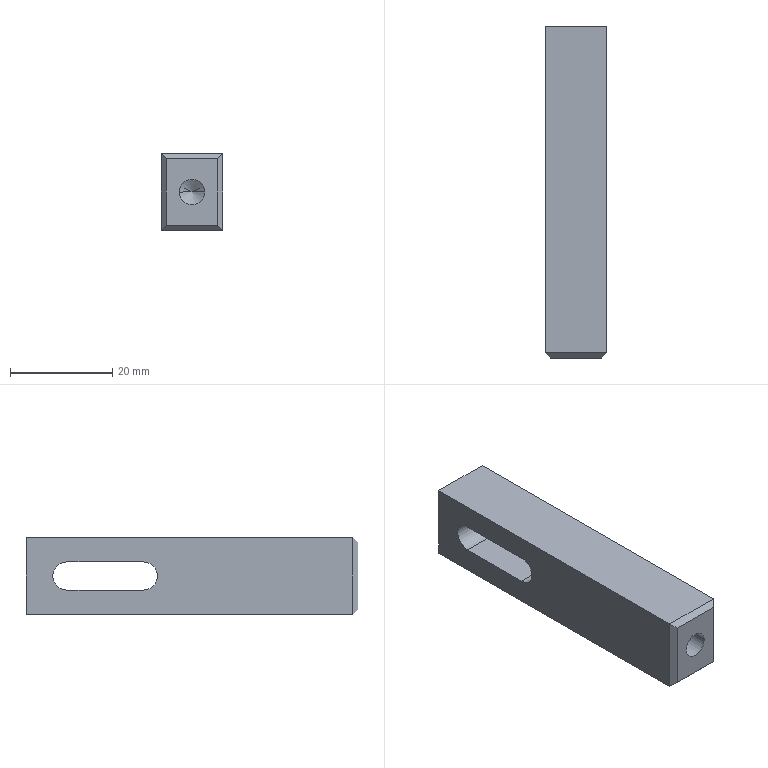Component | SolidWorks | ZL-10-02SupportPlate-1 | 1 solid | 18 faces | box 12 x 65 x 15 mm | volume 10095 mm3 | plane 12 | cylinder 4 | cone 2 | commonest cylinder face diameters 5 x2 5.5 x2
build123d program:
from build123d import *

# Parameters (mm, degrees)
SKETCH1_W             = 15
SKETCH1_H             = 65
EXTRUDE1_DEPTH        = 6
CUT_EXTRUDE1_DEPTH    = 67.523
M6_TAPPED_HOLE1_D     = 5
M6_TAPPED_HOLE1_DEPTH = 15
M6_TAPPED_HOLE1_TIP   = 1.502
CHAMFER1_SIZE         = 1


with BuildPart() as part:
    # Sketch1 → Extrude1 (new, symmetric)
    with BuildSketch(Plane.XY):
        with Locations((0, 32.5)):
            Rectangle(SKETCH1_W, SKETCH1_H)
    extrude(amount=EXTRUDE1_DEPTH, both=True)

    # Sketch2 → Cut-Extrude1 (cut, through all)
    with BuildSketch(Plane.XY.offset(6)):
        with BuildLine():
            Line((-2.75, 57), (-2.75, 42))
            ThreePointArc((-2.75, 42), (0, 39.25), (2.75, 42))
            Line((2.75, 42), (2.75, 57))
            ThreePointArc((2.75, 57), (0, 59.75), (-2.75, 57))
        make_face()
    extrude(amount=-CUT_EXTRUDE1_DEPTH, mode=Mode.SUBTRACT)

    # M6 Tapped Hole1
    with Locations(Plane.XZ):
        with Locations((0, 0)):
            Hole(M6_TAPPED_HOLE1_D / 2, depth=M6_TAPPED_HOLE1_DEPTH)
            with Locations((0, 0, -(M6_TAPPED_HOLE1_DEPTH + M6_TAPPED_HOLE1_TIP / 2))):  # 118° drill point
                Cone(0, M6_TAPPED_HOLE1_D / 2, M6_TAPPED_HOLE1_TIP, mode=Mode.SUBTRACT)

    # Chamfer1
    chamfer1_edges = [part.edges().sort_by_distance(p)[0] for p in [
        (0, 0, -6),
        (0, 0, 6),
        (7.5, 0, 0),
        (-7.5, 0, 0),
    ]]
    chamfer(chamfer1_edges, length=CHAMFER1_SIZE)


solid = part.part

# Placed as in the assembly
solid = solid.moved(Location((18.823, 6.749, -17), (0, 90, 0)))